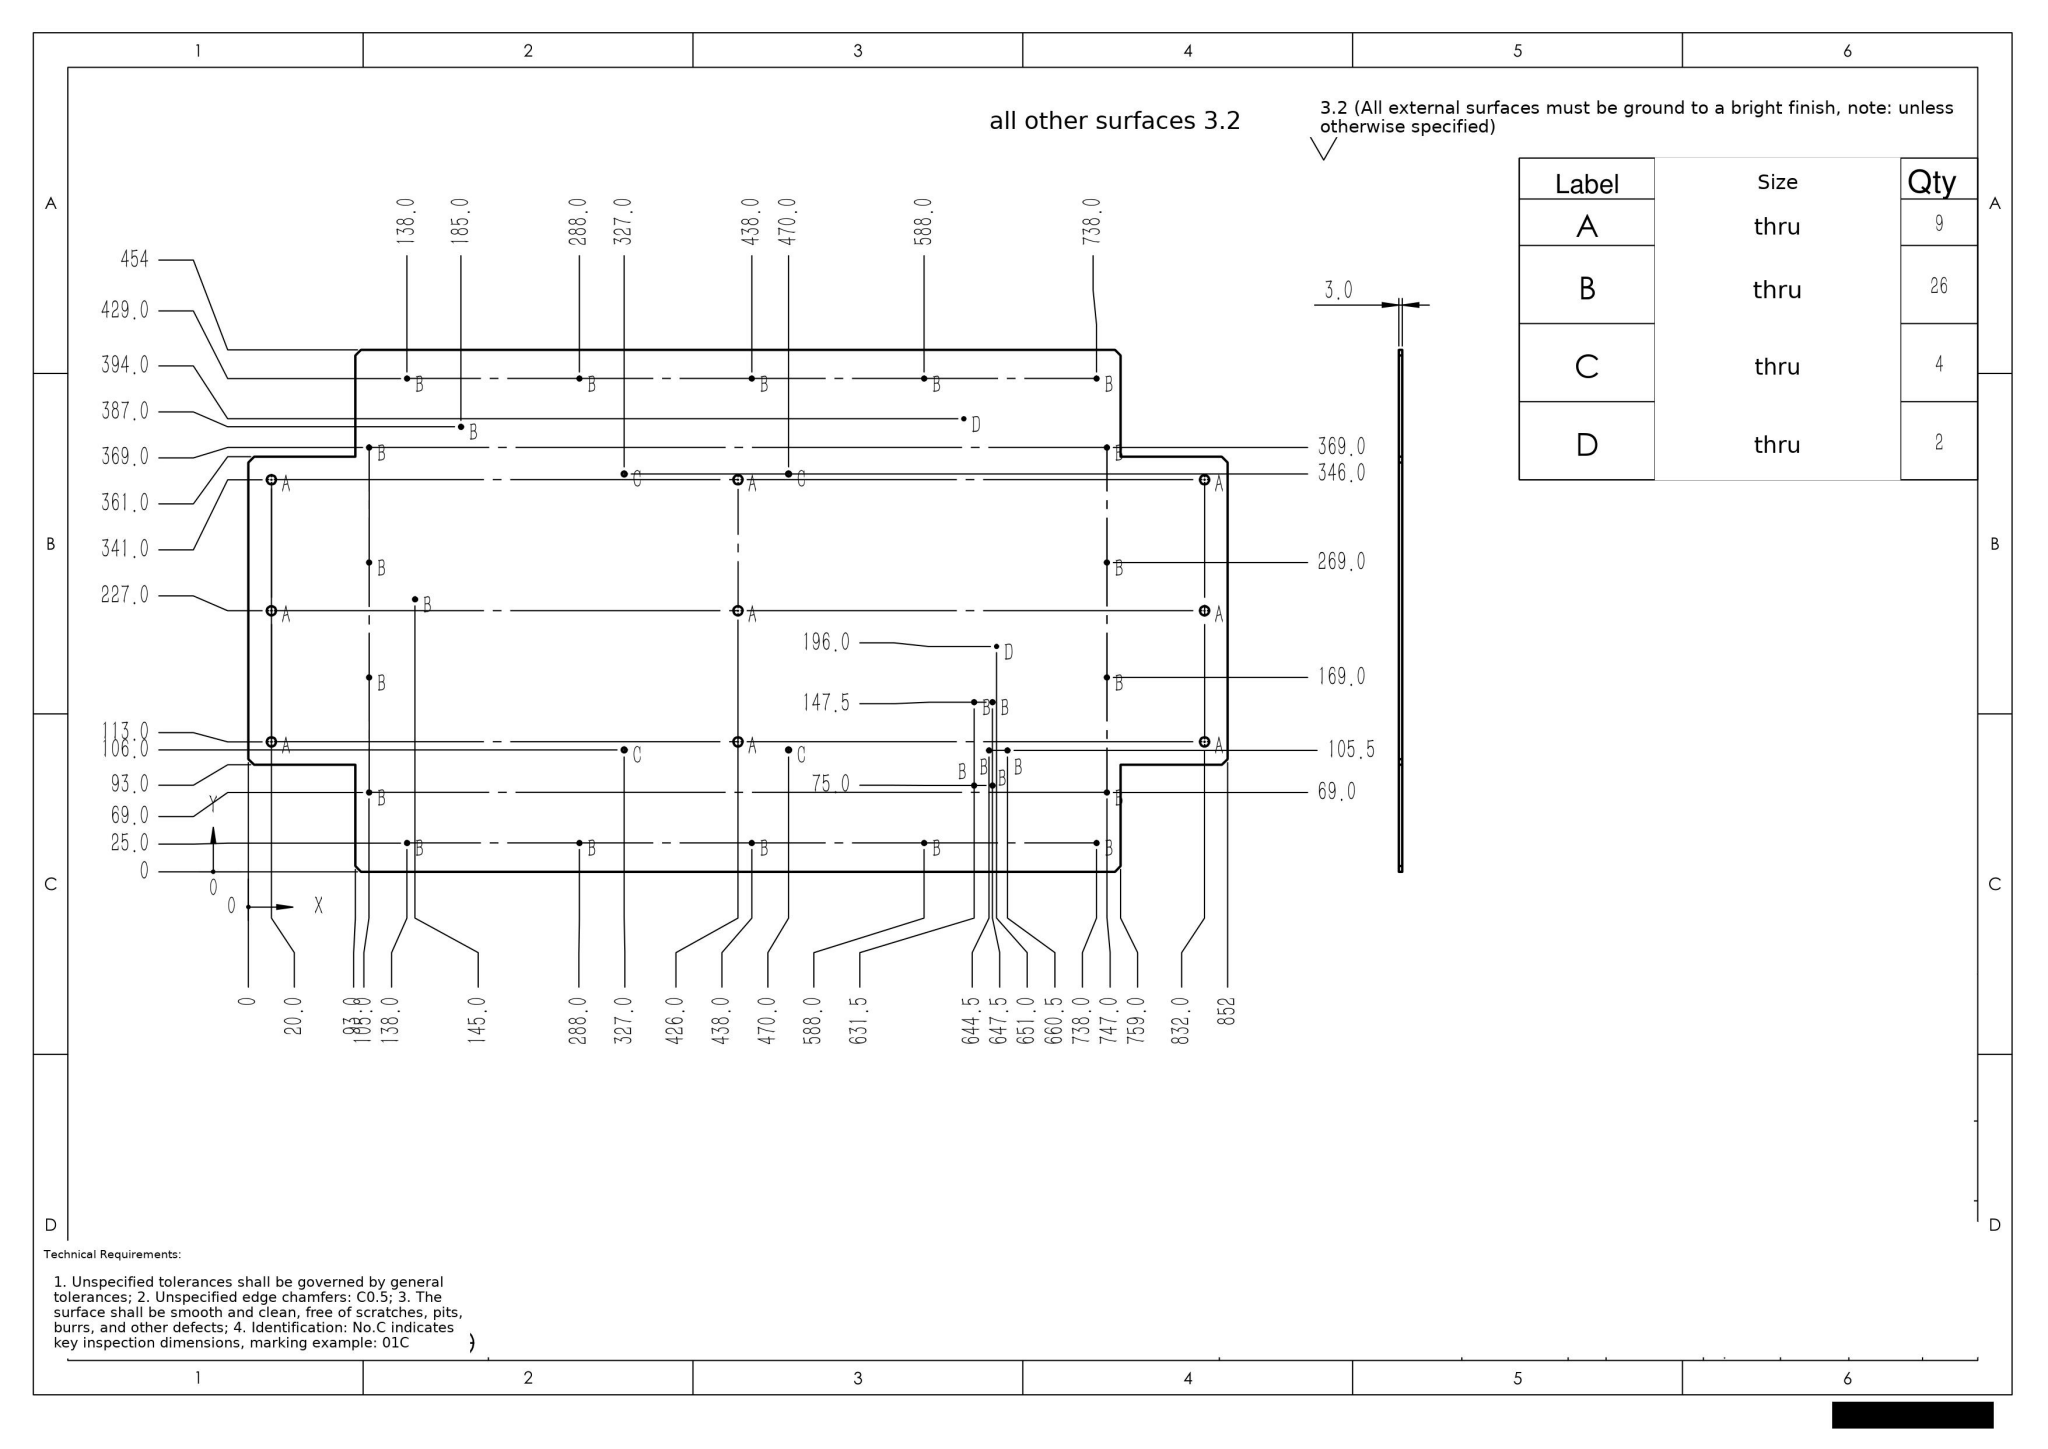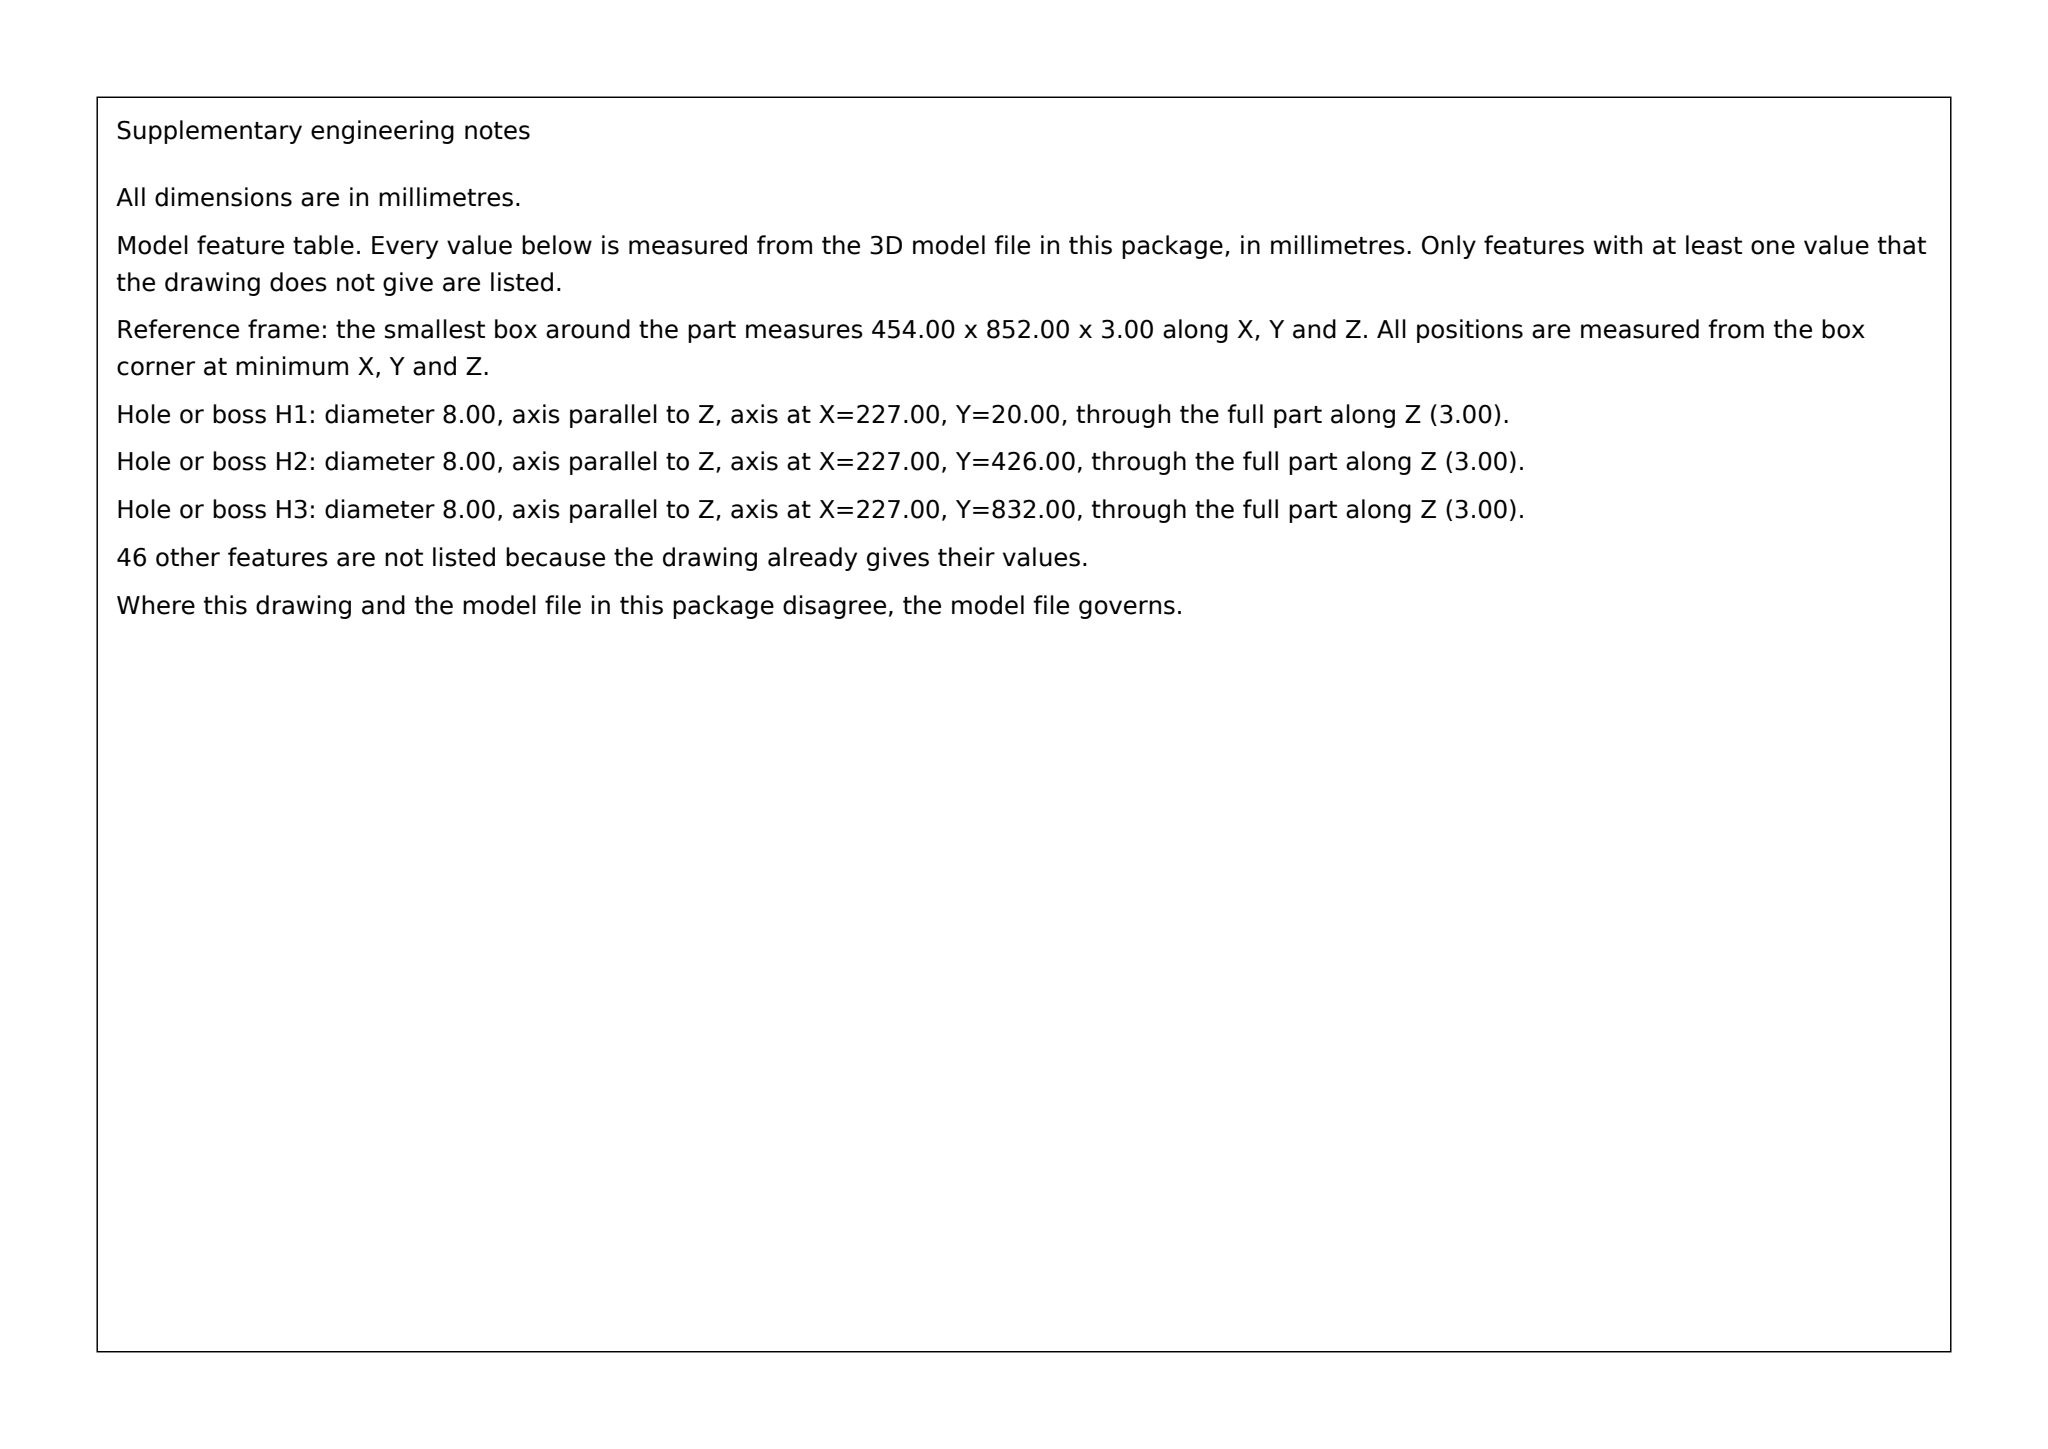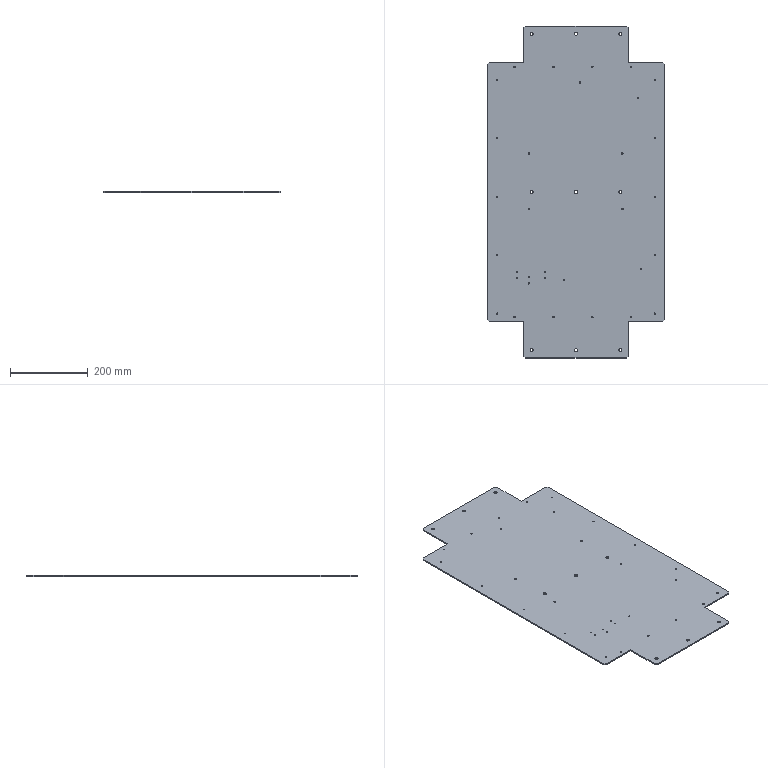Part | SolidWorks | mm | 1 solid | 104 faces | box 454 x 852 x 3 mm | volume 1054116 mm3 | cylinder 82 | plane 22 | commonest cylinder face diameters 3.3 x52 8 x18 4.2 x8 2.5 x4
build123d program:
from build123d import *

# Parameters (mm, degrees)
SKETCH1_W                = 454
SKETCH1_H                = 852
BOSS_EXTRUDE1_DEPTH      = 3
SKETCH2_W                = 93
SKETCH2_H                = 93
CUT_EXTRUDE1_DEPTH       = 483.715
F_8_0_8_DIAMETER_HOLE1_D = 8
CHAMFER1_SIZE            = 5
M4_TAPPED_HOLE1_D        = 3.3
LPATTERN1_COUNT          = 5
LPATTERN1_PITCH          = 150
M4_TAPPED_HOLE2_D        = 3.3
LPATTERN2_COUNT          = 4
LPATTERN2_PITCH          = 100
M5_TAPPED_HOLE1_D        = 4.2
M5_TAPPED_HOLE2_D        = 4.2
M4_TAPPED_HOLE3_D        = 3.3
M3_TAPPED_HOLE1_D        = 2.5
M4_TAPPED_HOLE4_D        = 3.3
M4_TAPPED_HOLE5_D        = 3.3


with BuildPart() as part:
    # Sketch1 → Boss-Extrude1 (new body)
    with BuildSketch(Plane.XY):
        Rectangle(SKETCH1_W, SKETCH1_H)
    extrude(amount=BOSS_EXTRUDE1_DEPTH)

    # Sketch2 → Cut-Extrude1 (cut, through all)
    with BuildSketch(Plane.XY.offset(3)):
        with Locations((-180.5, 379.5)):
            Rectangle(SKETCH2_W, SKETCH2_H)
        with Locations((-180.5, -379.5)):
            Rectangle(SKETCH2_W, SKETCH2_H)
        with Locations((180.5, -379.5)):
            Rectangle(SKETCH2_W, SKETCH2_H)
        with Locations((180.5, 379.5)):
            Rectangle(SKETCH2_W, SKETCH2_H)
    extrude(amount=-CUT_EXTRUDE1_DEPTH, mode=Mode.SUBTRACT)

    # 8.0 _8_ Diameter Hole1 (through all)
    with Locations(Plane.XY.offset(3)):
        with Locations((114, 406), (114, -406), (-114, -406), (-114, 406), (-114, 0), (114, 0), (0, 406), (0, -406), (0, 0)):
            Hole(F_8_0_8_DIAMETER_HOLE1_D / 2)

    # Chamfer1
    chamfer1_edges = [part.edges().sort_by_distance(p)[0] for p in [
        (-227, 333, 1.5),
        (-134, 426, 1.5),
        (-227, -333, 1.5),
        (-134, -426, 1.5),
        (227, -333, 1.5),
        (134, -426, 1.5),
        (227, 333, 1.5),
        (134, 426, 1.5),
    ]]
    chamfer(chamfer1_edges, length=CHAMFER1_SIZE)

    # M4 Tapped Hole1 (through all)
    with Locations(Plane.XY.offset(3)):
        with Locations((202, 288), (-202, 288)):
            m4_tapped_hole1 = Hole(M4_TAPPED_HOLE1_D / 2)

    # LPattern1: M4 Tapped Hole1 ×5
    with Locations(*[(0, -i * LPATTERN1_PITCH, 0) for i in range(1, LPATTERN1_COUNT)]):
        add(m4_tapped_hole1, mode=Mode.SUBTRACT)

    # M4 Tapped Hole2 (through all)
    with Locations(Plane.XY.offset(3)):
        with Locations((142, -321), (142, 321)):
            m4_tapped_hole2 = Hole(M4_TAPPED_HOLE2_D / 2)

    # LPattern2: M4 Tapped Hole2 ×4
    with Locations(*[(-i * LPATTERN2_PITCH, 0, 0) for i in range(1, LPATTERN2_COUNT)]):
        add(m4_tapped_hole2, mode=Mode.SUBTRACT)

    # M5 Tapped Hole1 (through all)
    with Locations(Plane.XY.offset(3)):
        with Locations((119, -44), (-121, -44)):
            Hole(M5_TAPPED_HOLE1_D / 2)

    # M5 Tapped Hole2 (through all)
    with Locations(Plane.XY.offset(3)):
        with Locations((119, 99), (-121, 99)):
            Hole(M5_TAPPED_HOLE2_D / 2)

    # M4 Tapped Hole3 (through all)
    with Locations(Plane.XY.offset(3)):
        with Locations((-152, -221.5), (-152, -205.5), (-79.5, -221.5), (-79.5, -205.5)):
            Hole(M4_TAPPED_HOLE3_D / 2)

    # M3 Tapped Hole1 (through all)
    with Locations(Plane.XY.offset(3)):
        with Locations((167, -196.5), (-31, -225)):
            Hole(M3_TAPPED_HOLE1_D / 2)

    # M4 Tapped Hole4 (through all)
    with Locations(Plane.XY.offset(3)):
        with Locations((160, 241), (10, 281)):
            Hole(M4_TAPPED_HOLE4_D / 2)

    # M4 Tapped Hole5 (through all)
    with Locations(Plane.XY.offset(3)):
        with Locations((-121.5, -218.5), (-121.5, -234.5)):
            Hole(M4_TAPPED_HOLE5_D / 2)


solid = part.part